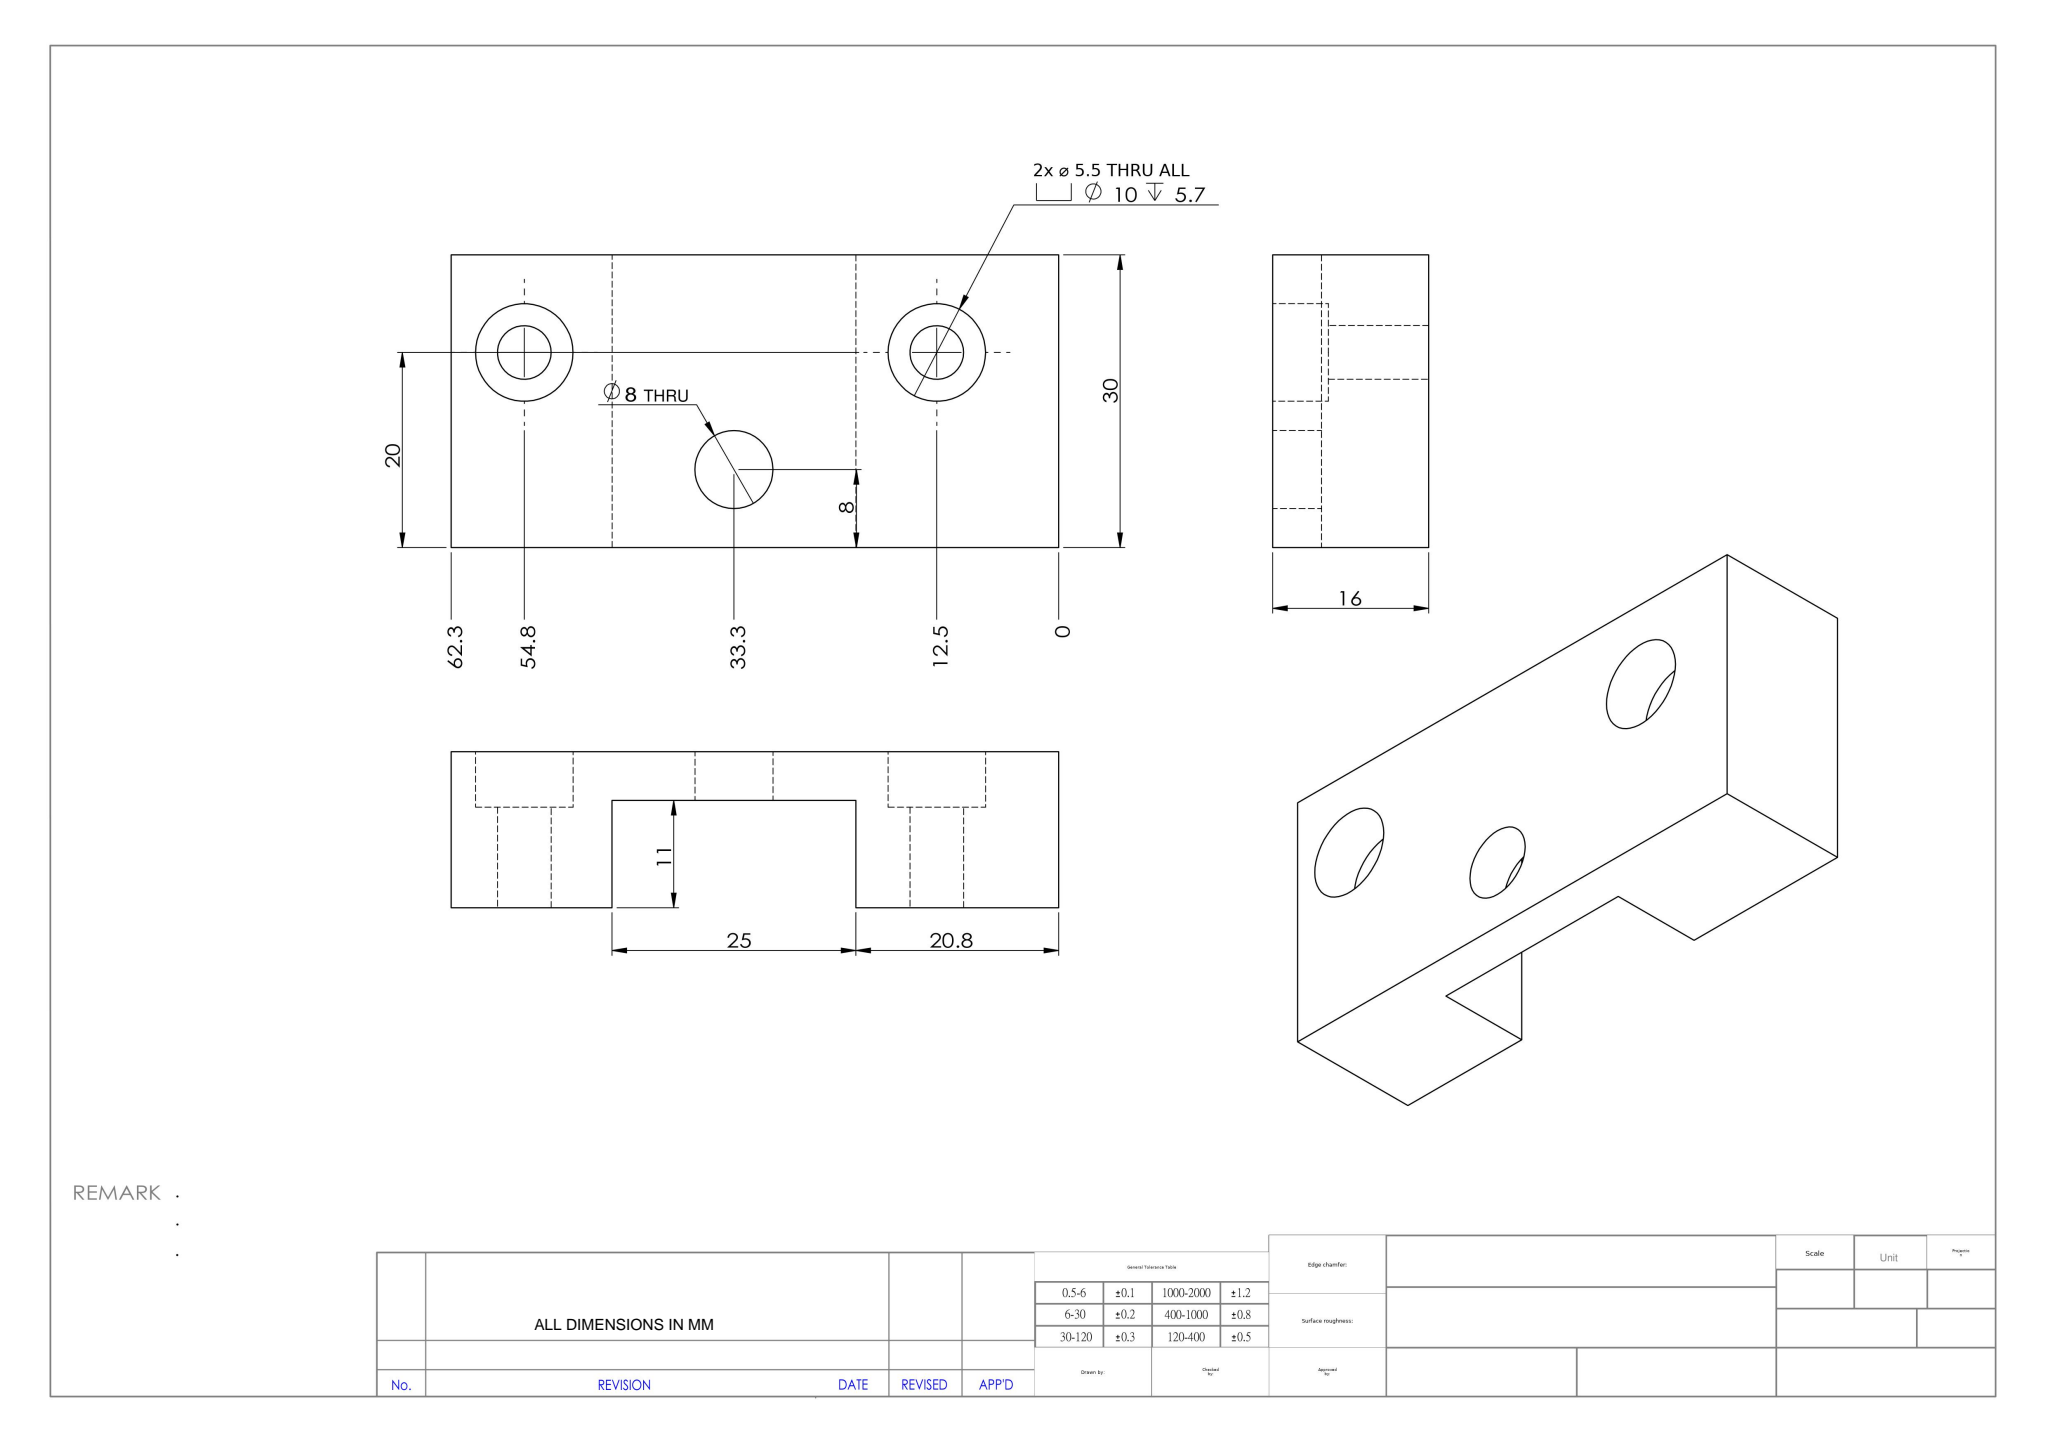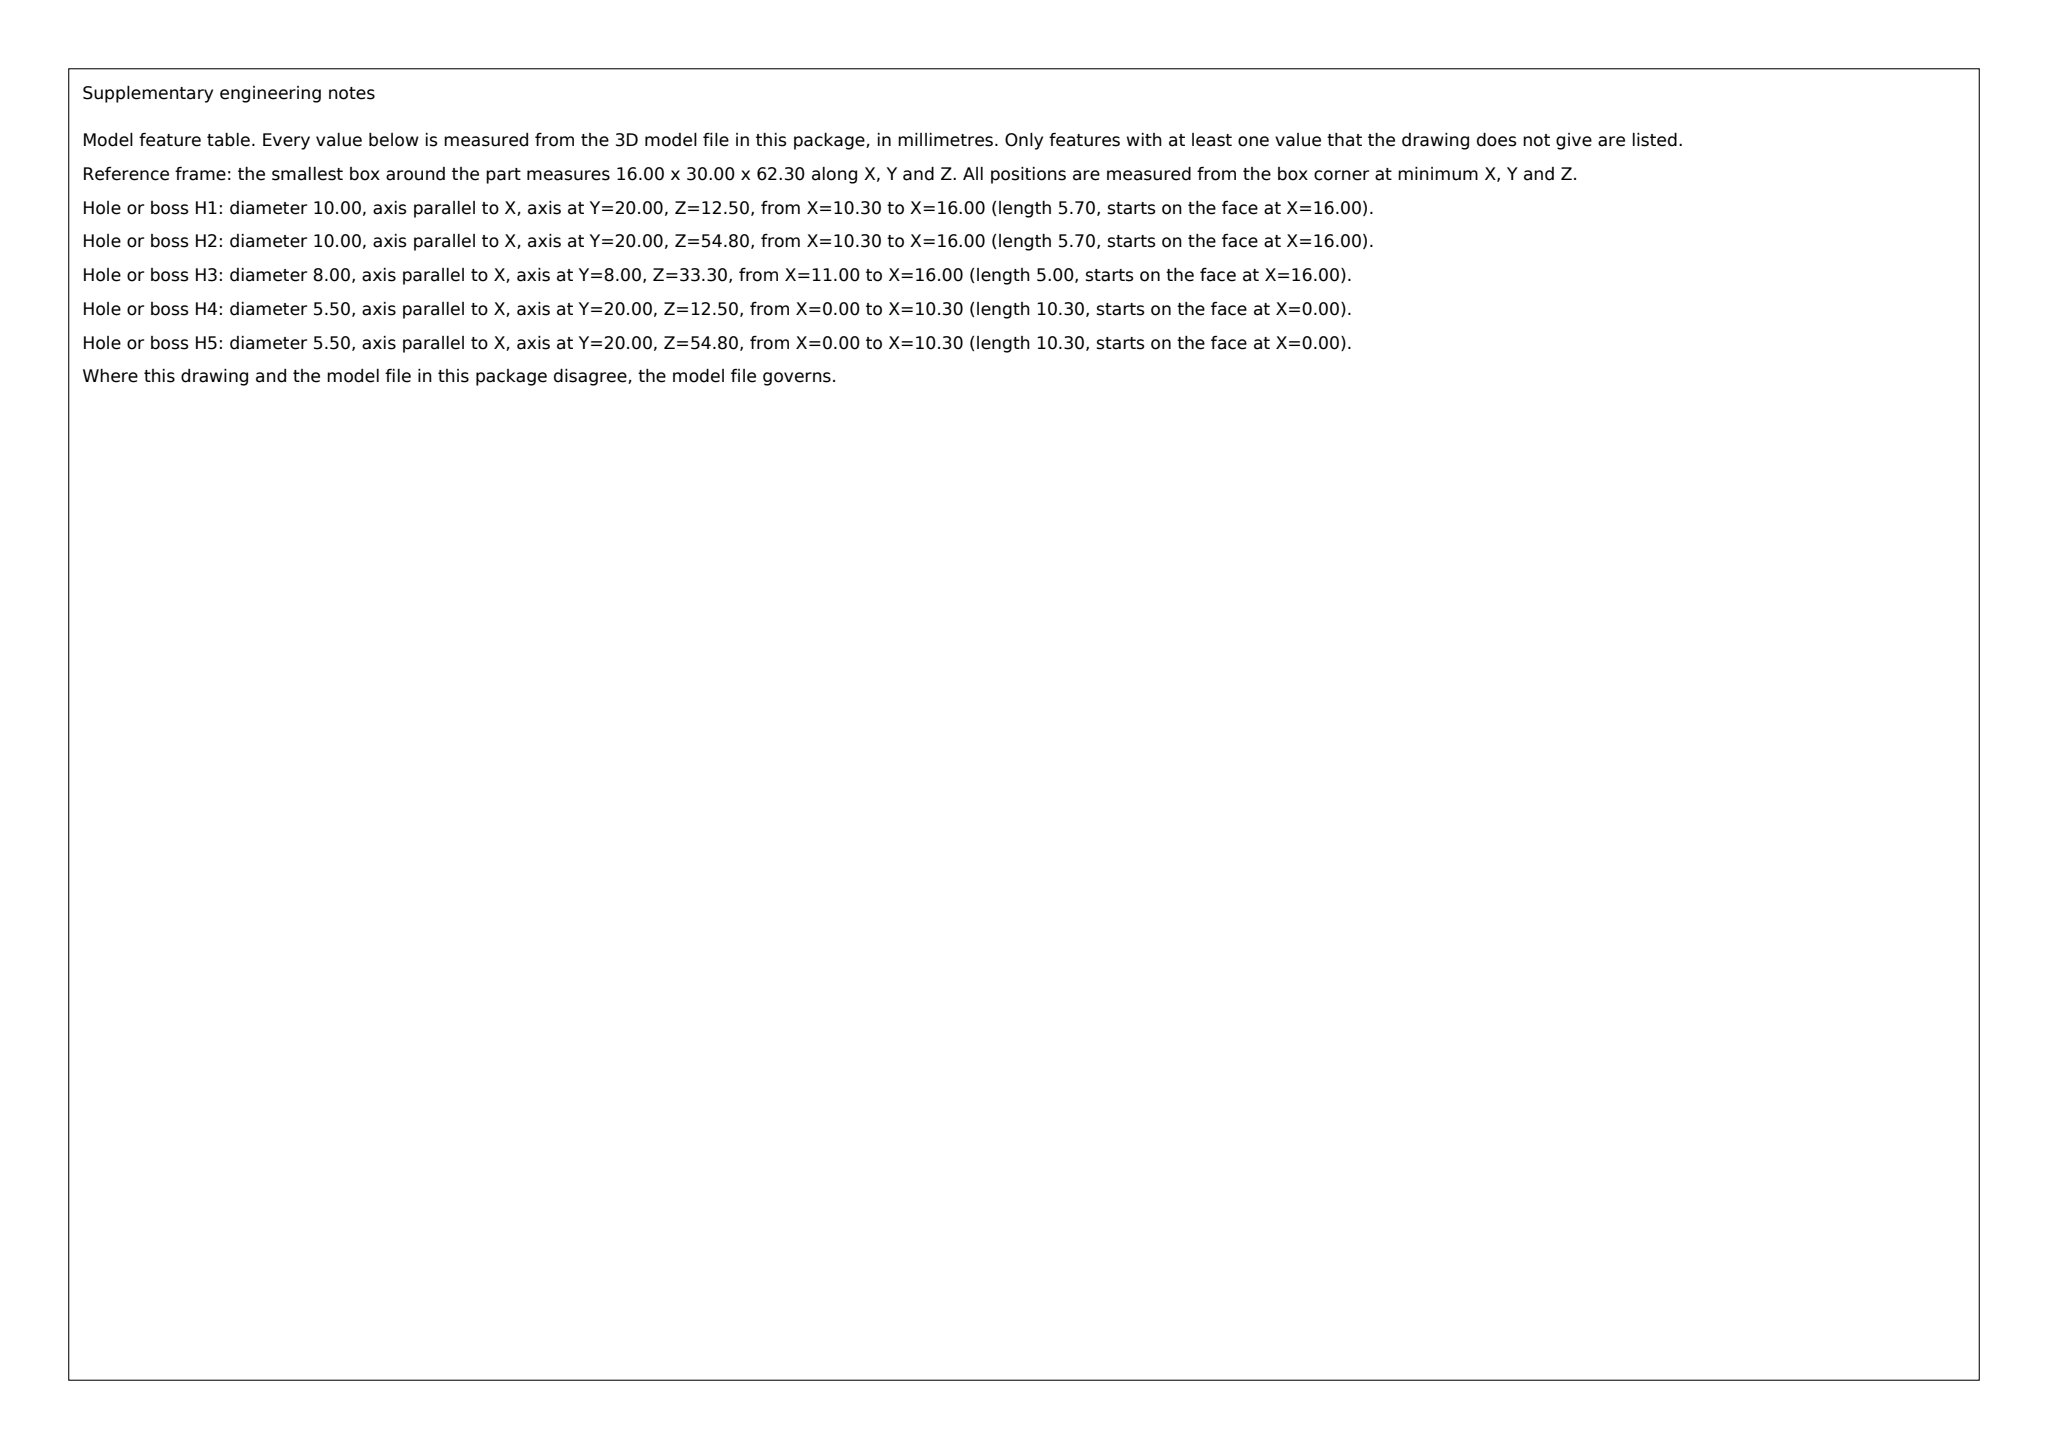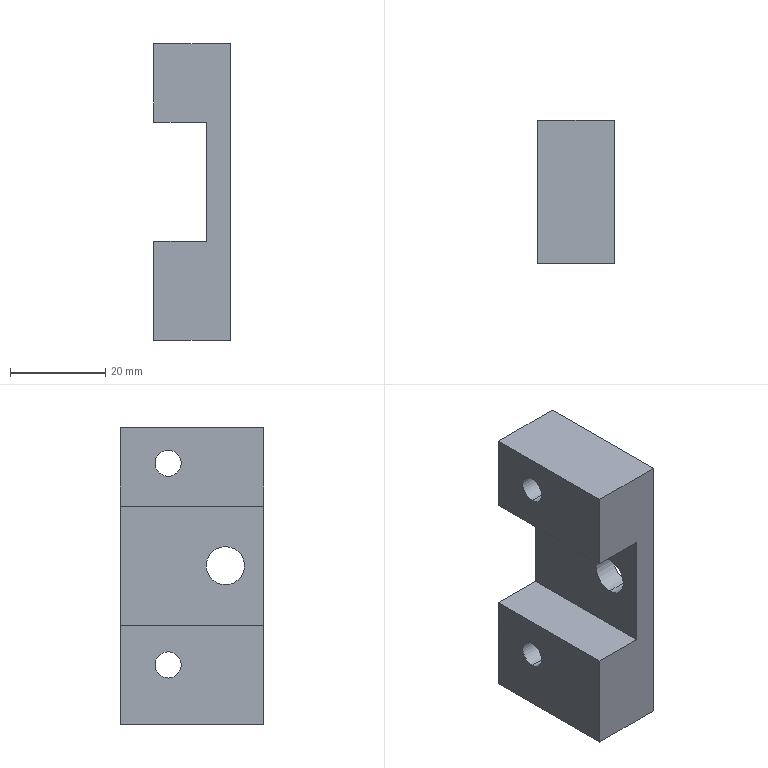Part | SolidWorks | mm | 1 solid | 22 faces | box 16 x 30 x 62.3 mm | volume 20018 mm3 | plane 12 | cylinder 10 | commonest cylinder face diameters 10 x4 5.5 x4 8 x2
build123d program:
from build123d import *

# Parameters (mm, degrees)
SKETCH1_W                                         = 62.3
SKETCH1_H                                         = 20
BOSS_EXTRUDE1_DEPTH                               = 16
HOLE_SIZE_ACCORDING_TO_TYPE_1_HEXAGON_D           = 5.5
HOLE_SIZE_ACCORDING_TO_TYPE_1_HEXAGON_CBORE_D     = 10
HOLE_SIZE_ACCORDING_TO_TYPE_1_HEXAGON_CBORE_DEPTH = 5.7
SKETCH5_W                                         = 16
SKETCH5_H                                         = 62.3
BOSS_EXTRUDE2_DEPTH                               = 10
SKETCH6_R                                         = 4
CUT_EXTRUDE1_DEPTH                                = 41.328
SKETCH7_W                                         = 25
SKETCH7_H                                         = 30
CUT_EXTRUDE2_DEPTH                                = 11


with BuildPart() as part:
    # Sketch1 → Boss-Extrude1 (new body)
    with BuildSketch(Plane(origin=(0, 0, 0), x_dir=(0, 0, -1), z_dir=(1, 0, 0))):
        Rectangle(SKETCH1_W, SKETCH1_H)
    extrude(amount=BOSS_EXTRUDE1_DEPTH)

    # Hole Size _ according to_ Type 1 Hexagon (through all)
    with Locations(Plane(origin=(16, 0, 0), x_dir=(0, 0, -1), z_dir=(1, 0, 0))):
        with Locations((-23.65, 0), (18.65, 0)):
            CounterBoreHole(HOLE_SIZE_ACCORDING_TO_TYPE_1_HEXAGON_D / 2, HOLE_SIZE_ACCORDING_TO_TYPE_1_HEXAGON_CBORE_D / 2, HOLE_SIZE_ACCORDING_TO_TYPE_1_HEXAGON_CBORE_DEPTH)

    # Sketch5 → Boss-Extrude2 (add)
    with BuildSketch(Plane.XZ.offset(10)):
        with Locations((8, 0)):
            Rectangle(SKETCH5_W, SKETCH5_H)
    extrude(amount=BOSS_EXTRUDE2_DEPTH)

    # Sketch6 → Cut-Extrude1 (cut, through all)
    with BuildSketch(Plane(origin=(16, 0, 0), x_dir=(0, 0, -1), z_dir=(1, 0, 0))):
        with Locations((-2.15, -12)):
            Circle(SKETCH6_R)
    extrude(amount=-CUT_EXTRUDE1_DEPTH, mode=Mode.SUBTRACT)

    # Sketch7 → Cut-Extrude2 (cut)
    with BuildSketch(Plane.ZY):
        with Locations((2.15, -5)):
            Rectangle(SKETCH7_W, SKETCH7_H)
    extrude(amount=-CUT_EXTRUDE2_DEPTH, mode=Mode.SUBTRACT)


solid = part.part
STEP:
#1=CARTESIAN_POINT('',(11.,-12.,-1.85));
#2=VERTEX_POINT('',#1);
#3=CARTESIAN_POINT('',(11.,-12.,6.15));
#4=VERTEX_POINT('',#3);
#5=CARTESIAN_POINT('',(11.,-12.,2.15));
#6=DIRECTION('',(-1.,0.,0.));
#7=DIRECTION('',(0.,0.,-1.));
#8=AXIS2_PLACEMENT_3D('',#5,#6,#7);
#9=CIRCLE('',#8,4.);
#10=EDGE_CURVE('',#2,#4,#9,.T.);
#11=ORIENTED_EDGE('',*,*,#10,.T.);
#12=CARTESIAN_POINT('',(16.,-12.,6.15));
#13=VERTEX_POINT('',#12);
#14=CARTESIAN_POINT('',(0.,-12.,6.15));
#15=DIRECTION('',(1.,0.,0.));
#16=VECTOR('',#15,1000.);
#17=LINE('',#14,#16);
#18=EDGE_CURVE('',#4,#13,#17,.T.);
#19=ORIENTED_EDGE('',*,*,#18,.T.);
#20=CARTESIAN_POINT('',(16.,-12.,-1.85));
#21=VERTEX_POINT('',#20);
#22=CARTESIAN_POINT('',(16.,-12.,2.15));
#23=DIRECTION('',(1.,0.,0.));
#24=DIRECTION('',(0.,0.,-1.));
#25=AXIS2_PLACEMENT_3D('',#22,#23,#24);
#26=CIRCLE('',#25,4.);
#27=EDGE_CURVE('',#13,#21,#26,.T.);
#28=ORIENTED_EDGE('',*,*,#27,.T.);
#29=CARTESIAN_POINT('',(0.,-12.,-1.85));
#30=DIRECTION('',(1.,0.,0.));
#31=VECTOR('',#30,1000.);
#32=LINE('',#29,#31);
#33=EDGE_CURVE('',#2,#21,#32,.T.);
#34=ORIENTED_EDGE('',*,*,#33,.F.);
#35=EDGE_LOOP('',(#11,#19,#28,#34));
#36=FACE_OUTER_BOUND('',#35,.T.);
#37=CARTESIAN_POINT('',(0.,-12.,2.15));
#38=DIRECTION('',(1.,0.,0.));
#39=DIRECTION('',(0.,0.,-1.));
#40=AXIS2_PLACEMENT_3D('',#37,#38,#39);
#41=CYLINDRICAL_SURFACE('',#40,4.);
#42=ADVANCED_FACE('',(#36),#41,.F.);
#43=CARTESIAN_POINT('',(10.3,0.,28.65));
#44=VERTEX_POINT('',#43);
#45=CARTESIAN_POINT('',(10.3,0.,18.65));
#46=VERTEX_POINT('',#45);
#47=CARTESIAN_POINT('',(10.3,0.,23.65));
#48=DIRECTION('',(1.,0.,0.));
#49=DIRECTION('',(0.,0.,-1.));
#50=AXIS2_PLACEMENT_3D('',#47,#48,#49);
#51=CIRCLE('',#50,5.);
#52=EDGE_CURVE('',#44,#46,#51,.T.);
#53=ORIENTED_EDGE('',*,*,#52,.F.);
#54=CARTESIAN_POINT('',(16.,0.,28.65));
#55=VERTEX_POINT('',#54);
#56=CARTESIAN_POINT('',(16.,0.,28.65));
#57=DIRECTION('',(1.,0.,0.));
#58=VECTOR('',#57,1000.);
#59=LINE('',#56,#58);
#60=EDGE_CURVE('',#44,#55,#59,.T.);
#61=ORIENTED_EDGE('',*,*,#60,.T.);
#62=CARTESIAN_POINT('',(16.,0.,18.65));
#63=VERTEX_POINT('',#62);
#64=CARTESIAN_POINT('',(16.,0.,23.65));
#65=DIRECTION('',(1.,0.,0.));
#66=DIRECTION('',(0.,0.,-1.));
#67=AXIS2_PLACEMENT_3D('',#64,#65,#66);
#68=CIRCLE('',#67,5.);
#69=EDGE_CURVE('',#55,#63,#68,.T.);
#70=ORIENTED_EDGE('',*,*,#69,.T.);
#71=CARTESIAN_POINT('',(16.,0.,18.65));
#72=DIRECTION('',(1.,0.,0.));
#73=VECTOR('',#72,1000.);
#74=LINE('',#71,#73);
#75=EDGE_CURVE('',#46,#63,#74,.T.);
#76=ORIENTED_EDGE('',*,*,#75,.F.);
#77=EDGE_LOOP('',(#53,#61,#70,#76));
#78=FACE_OUTER_BOUND('',#77,.T.);
#79=CARTESIAN_POINT('',(16.,0.,23.65));
#80=DIRECTION('',(1.,0.,0.));
#81=DIRECTION('',(0.,0.,-1.));
#82=AXIS2_PLACEMENT_3D('',#79,#80,#81);
#83=CYLINDRICAL_SURFACE('',#82,5.);
#84=ADVANCED_FACE('',(#78),#83,.F.);
#85=CARTESIAN_POINT('',(0.,0.,26.4));
#86=VERTEX_POINT('',#85);
#87=CARTESIAN_POINT('',(0.,0.,20.9));
#88=VERTEX_POINT('',#87);
#89=CARTESIAN_POINT('',(0.,0.,23.65));
#90=DIRECTION('',(1.,0.,0.));
#91=DIRECTION('',(0.,0.,-1.));
#92=AXIS2_PLACEMENT_3D('',#89,#90,#91);
#93=CIRCLE('',#92,2.75);
#94=EDGE_CURVE('',#86,#88,#93,.T.);
#95=ORIENTED_EDGE('',*,*,#94,.F.);
#96=CARTESIAN_POINT('',(10.3,0.,26.4));
#97=VERTEX_POINT('',#96);
#98=CARTESIAN_POINT('',(16.,0.,26.4));
#99=DIRECTION('',(1.,0.,0.));
#100=VECTOR('',#99,1000.);
#101=LINE('',#98,#100);
#102=EDGE_CURVE('',#86,#97,#101,.T.);
#103=ORIENTED_EDGE('',*,*,#102,.T.);
#104=CARTESIAN_POINT('',(10.3,0.,20.9));
#105=VERTEX_POINT('',#104);
#106=CARTESIAN_POINT('',(10.3,0.,23.65));
#107=DIRECTION('',(1.,0.,0.));
#108=DIRECTION('',(0.,0.,-1.));
#109=AXIS2_PLACEMENT_3D('',#106,#107,#108);
#110=CIRCLE('',#109,2.75);
#111=EDGE_CURVE('',#97,#105,#110,.T.);
#112=ORIENTED_EDGE('',*,*,#111,.T.);
#113=CARTESIAN_POINT('',(16.,0.,20.9));
#114=DIRECTION('',(1.,0.,0.));
#115=VECTOR('',#114,1000.);
#116=LINE('',#113,#115);
#117=EDGE_CURVE('',#88,#105,#116,.T.);
#118=ORIENTED_EDGE('',*,*,#117,.F.);
#119=EDGE_LOOP('',(#95,#103,#112,#118));
#120=FACE_OUTER_BOUND('',#119,.T.);
#121=CARTESIAN_POINT('',(16.,0.,23.65));
#122=DIRECTION('',(1.,0.,0.));
#123=DIRECTION('',(0.,0.,-1.));
#124=AXIS2_PLACEMENT_3D('',#121,#122,#123);
#125=CYLINDRICAL_SURFACE('',#124,2.75);
#126=ADVANCED_FACE('',(#120),#125,.F.);
#127=CARTESIAN_POINT('',(10.3,0.,-13.65));
#128=VERTEX_POINT('',#127);
#129=CARTESIAN_POINT('',(10.3,0.,-23.65));
#130=VERTEX_POINT('',#129);
#131=CARTESIAN_POINT('',(10.3,0.,-18.65));
#132=DIRECTION('',(1.,0.,0.));
#133=DIRECTION('',(0.,0.,-1.));
#134=AXIS2_PLACEMENT_3D('',#131,#132,#133);
#135=CIRCLE('',#134,5.);
#136=EDGE_CURVE('',#128,#130,#135,.T.);
#137=ORIENTED_EDGE('',*,*,#136,.F.);
#138=CARTESIAN_POINT('',(16.,0.,-13.65));
#139=VERTEX_POINT('',#138);
#140=CARTESIAN_POINT('',(16.,0.,-13.65));
#141=DIRECTION('',(1.,0.,0.));
#142=VECTOR('',#141,1000.);
#143=LINE('',#140,#142);
#144=EDGE_CURVE('',#128,#139,#143,.T.);
#145=ORIENTED_EDGE('',*,*,#144,.T.);
#146=CARTESIAN_POINT('',(16.,0.,-23.65));
#147=VERTEX_POINT('',#146);
#148=CARTESIAN_POINT('',(16.,0.,-18.65));
#149=DIRECTION('',(1.,0.,0.));
#150=DIRECTION('',(0.,0.,-1.));
#151=AXIS2_PLACEMENT_3D('',#148,#149,#150);
#152=CIRCLE('',#151,5.);
#153=EDGE_CURVE('',#139,#147,#152,.T.);
#154=ORIENTED_EDGE('',*,*,#153,.T.);
#155=CARTESIAN_POINT('',(16.,0.,-23.65));
#156=DIRECTION('',(1.,0.,0.));
#157=VECTOR('',#156,1000.);
#158=LINE('',#155,#157);
#159=EDGE_CURVE('',#130,#147,#158,.T.);
#160=ORIENTED_EDGE('',*,*,#159,.F.);
#161=EDGE_LOOP('',(#137,#145,#154,#160));
#162=FACE_OUTER_BOUND('',#161,.T.);
#163=CARTESIAN_POINT('',(16.,0.,-18.65));
#164=DIRECTION('',(1.,0.,0.));
#165=DIRECTION('',(0.,0.,-1.));
#166=AXIS2_PLACEMENT_3D('',#163,#164,#165);
#167=CYLINDRICAL_SURFACE('',#166,5.);
#168=ADVANCED_FACE('',(#162),#167,.F.);
#169=CARTESIAN_POINT('',(0.,0.,-15.9));
#170=VERTEX_POINT('',#169);
#171=CARTESIAN_POINT('',(0.,0.,-21.4));
#172=VERTEX_POINT('',#171);
#173=CARTESIAN_POINT('',(0.,0.,-18.65));
#174=DIRECTION('',(1.,0.,0.));
#175=DIRECTION('',(0.,0.,-1.));
#176=AXIS2_PLACEMENT_3D('',#173,#174,#175);
#177=CIRCLE('',#176,2.75);
#178=EDGE_CURVE('',#170,#172,#177,.T.);
#179=ORIENTED_EDGE('',*,*,#178,.F.);
#180=CARTESIAN_POINT('',(10.3,0.,-15.9));
#181=VERTEX_POINT('',#180);
#182=CARTESIAN_POINT('',(16.,0.,-15.9));
#183=DIRECTION('',(1.,0.,0.));
#184=VECTOR('',#183,1000.);
#185=LINE('',#182,#184);
#186=EDGE_CURVE('',#170,#181,#185,.T.);
#187=ORIENTED_EDGE('',*,*,#186,.T.);
#188=CARTESIAN_POINT('',(10.3,0.,-21.4));
#189=VERTEX_POINT('',#188);
#190=CARTESIAN_POINT('',(10.3,0.,-18.65));
#191=DIRECTION('',(1.,0.,0.));
#192=DIRECTION('',(0.,0.,-1.));
#193=AXIS2_PLACEMENT_3D('',#190,#191,#192);
#194=CIRCLE('',#193,2.75);
#195=EDGE_CURVE('',#181,#189,#194,.T.);
#196=ORIENTED_EDGE('',*,*,#195,.T.);
#197=CARTESIAN_POINT('',(16.,0.,-21.4));
#198=DIRECTION('',(1.,0.,0.));
#199=VECTOR('',#198,1000.);
#200=LINE('',#197,#199);
#201=EDGE_CURVE('',#172,#189,#200,.T.);
#202=ORIENTED_EDGE('',*,*,#201,.F.);
#203=EDGE_LOOP('',(#179,#187,#196,#202));
#204=FACE_OUTER_BOUND('',#203,.T.);
#205=CARTESIAN_POINT('',(16.,0.,-18.65));
#206=DIRECTION('',(1.,0.,0.));
#207=DIRECTION('',(0.,0.,-1.));
#208=AXIS2_PLACEMENT_3D('',#205,#206,#207);
#209=CYLINDRICAL_SURFACE('',#208,2.75);
#210=ADVANCED_FACE('',(#204),#209,.F.);
#211=CARTESIAN_POINT('',(0.,0.,-18.65));
#212=DIRECTION('',(1.,0.,0.));
#213=DIRECTION('',(0.,0.,-1.));
#214=AXIS2_PLACEMENT_3D('',#211,#212,#213);
#215=CIRCLE('',#214,2.75);
#216=EDGE_CURVE('',#172,#170,#215,.T.);
#217=ORIENTED_EDGE('',*,*,#216,.T.);
#218=ORIENTED_EDGE('',*,*,#178,.T.);
#219=EDGE_LOOP('',(#217,#218));
#220=FACE_BOUND('',#219,.T.);
#221=CARTESIAN_POINT('',(0.,-20.,-10.35));
#222=VERTEX_POINT('',#221);
#223=CARTESIAN_POINT('',(0.,-20.,-31.15));
#224=VERTEX_POINT('',#223);
#225=CARTESIAN_POINT('',(0.,-20.,31.15));
#226=DIRECTION('',(0.,0.,-1.));
#227=VECTOR('',#226,1000.);
#228=LINE('',#225,#227);
#229=EDGE_CURVE('',#222,#224,#228,.T.);
#230=ORIENTED_EDGE('',*,*,#229,.F.);
#231=CARTESIAN_POINT('',(0.,10.,-10.35));
#232=VERTEX_POINT('',#231);
#233=CARTESIAN_POINT('',(0.,-20.,-10.35));
#234=DIRECTION('',(0.,-1.,0.));
#235=VECTOR('',#234,1000.);
#236=LINE('',#233,#235);
#237=EDGE_CURVE('',#232,#222,#236,.T.);
#238=ORIENTED_EDGE('',*,*,#237,.F.);
#239=CARTESIAN_POINT('',(0.,10.,-31.15));
#240=VERTEX_POINT('',#239);
#241=CARTESIAN_POINT('',(0.,10.,-31.15));
#242=DIRECTION('',(0.,-0.,1.));
#243=VECTOR('',#242,1000.);
#244=LINE('',#241,#243);
#245=EDGE_CURVE('',#240,#232,#244,.T.);
#246=ORIENTED_EDGE('',*,*,#245,.F.);
#247=CARTESIAN_POINT('',(0.,-10.,-31.15));
#248=DIRECTION('',(0.,1.,0.));
#249=VECTOR('',#248,1000.);
#250=LINE('',#247,#249);
#251=EDGE_CURVE('',#224,#240,#250,.T.);
#252=ORIENTED_EDGE('',*,*,#251,.F.);
#253=EDGE_LOOP('',(#230,#238,#246,#252));
#254=FACE_OUTER_BOUND('',#253,.T.);
#255=CARTESIAN_POINT('',(0.,0.,0.));
#256=DIRECTION('',(1.,0.,0.));
#257=DIRECTION('',(0.,0.,-1.));
#258=AXIS2_PLACEMENT_3D('',#255,#256,#257);
#259=PLANE('',#258);
#260=ADVANCED_FACE('',(#220,#254),#259,.F.);
#261=CARTESIAN_POINT('',(0.,10.,31.15));
#262=VERTEX_POINT('',#261);
#263=CARTESIAN_POINT('',(0.,-20.,31.15));
#264=VERTEX_POINT('',#263);
#265=CARTESIAN_POINT('',(0.,-10.,31.15));
#266=DIRECTION('',(0.,-1.,0.));
#267=VECTOR('',#266,1000.);
#268=LINE('',#265,#267);
#269=EDGE_CURVE('',#262,#264,#268,.T.);
#270=ORIENTED_EDGE('',*,*,#269,.T.);
#271=CARTESIAN_POINT('',(16.,-20.,31.15));
#272=VERTEX_POINT('',#271);
#273=CARTESIAN_POINT('',(16.,-20.,31.15));
#274=DIRECTION('',(-1.,0.,0.));
#275=VECTOR('',#274,1000.);
#276=LINE('',#273,#275);
#277=EDGE_CURVE('',#272,#264,#276,.T.);
#278=ORIENTED_EDGE('',*,*,#277,.F.);
#279=CARTESIAN_POINT('',(16.,10.,31.15));
#280=VERTEX_POINT('',#279);
#281=CARTESIAN_POINT('',(16.,-10.,31.15));
#282=DIRECTION('',(0.,-1.,0.));
#283=VECTOR('',#282,1000.);
#284=LINE('',#281,#283);
#285=EDGE_CURVE('',#280,#272,#284,.T.);
#286=ORIENTED_EDGE('',*,*,#285,.F.);
#287=CARTESIAN_POINT('',(16.,10.,31.15));
#288=DIRECTION('',(-1.,0.,0.));
#289=VECTOR('',#288,1000.);
#290=LINE('',#287,#289);
#291=EDGE_CURVE('',#280,#262,#290,.T.);
#292=ORIENTED_EDGE('',*,*,#291,.T.);
#293=EDGE_LOOP('',(#270,#278,#286,#292));
#294=FACE_OUTER_BOUND('',#293,.T.);
#295=CARTESIAN_POINT('',(16.,-10.,31.15));
#296=DIRECTION('',(0.,0.,-1.));
#297=DIRECTION('',(-1.,0.,0.));
#298=AXIS2_PLACEMENT_3D('',#295,#296,#297);
#299=PLANE('',#298);
#300=ADVANCED_FACE('',(#294),#299,.F.);
#301=ORIENTED_EDGE('',*,*,#251,.T.);
#302=CARTESIAN_POINT('',(16.,10.,-31.15));
#303=VERTEX_POINT('',#302);
#304=CARTESIAN_POINT('',(16.,10.,-31.15));
#305=DIRECTION('',(-1.,0.,0.));
#306=VECTOR('',#305,1000.);
#307=LINE('',#304,#306);
#308=EDGE_CURVE('',#303,#240,#307,.T.);
#309=ORIENTED_EDGE('',*,*,#308,.F.);
#310=CARTESIAN_POINT('',(16.,-20.,-31.15));
#311=VERTEX_POINT('',#310);
#312=CARTESIAN_POINT('',(16.,-10.,-31.15));
#313=DIRECTION('',(0.,1.,0.));
#314=VECTOR('',#313,1000.);
#315=LINE('',#312,#314);
#316=EDGE_CURVE('',#311,#303,#315,.T.);
#317=ORIENTED_EDGE('',*,*,#316,.F.);
#318=CARTESIAN_POINT('',(0.,-20.,-31.15));
#319=DIRECTION('',(1.,0.,0.));
#320=VECTOR('',#319,1000.);
#321=LINE('',#318,#320);
#322=EDGE_CURVE('',#224,#311,#321,.T.);
#323=ORIENTED_EDGE('',*,*,#322,.F.);
#324=EDGE_LOOP('',(#301,#309,#317,#323));
#325=FACE_OUTER_BOUND('',#324,.T.);
#326=CARTESIAN_POINT('',(16.,-10.,-31.15));
#327=DIRECTION('',(0.,0.,1.));
#328=DIRECTION('',(1.,0.,0.));
#329=AXIS2_PLACEMENT_3D('',#326,#327,#328);
#330=PLANE('',#329);
#331=ADVANCED_FACE('',(#325),#330,.F.);
#332=ORIENTED_EDGE('',*,*,#245,.T.);
#333=CARTESIAN_POINT('',(11.,10.,-10.35));
#334=VERTEX_POINT('',#333);
#335=CARTESIAN_POINT('',(11.,10.,-10.35));
#336=DIRECTION('',(-1.,0.,0.));
#337=VECTOR('',#336,1000.);
#338=LINE('',#335,#337);
#339=EDGE_CURVE('',#334,#232,#338,.T.);
#340=ORIENTED_EDGE('',*,*,#339,.F.);
#341=CARTESIAN_POINT('',(11.,10.,14.65));
#342=VERTEX_POINT('',#341);
#343=CARTESIAN_POINT('',(11.,10.,-10.35));
#344=DIRECTION('',(0.,0.,-1.));
#345=VECTOR('',#344,1000.);
#346=LINE('',#343,#345);
#347=EDGE_CURVE('',#342,#334,#346,.T.);
#348=ORIENTED_EDGE('',*,*,#347,.F.);
#349=CARTESIAN_POINT('',(0.,10.,14.65));
#350=VERTEX_POINT('',#349);
#351=CARTESIAN_POINT('',(11.,10.,14.65));
#352=DIRECTION('',(-1.,0.,0.));
#353=VECTOR('',#352,1000.);
#354=LINE('',#351,#353);
#355=EDGE_CURVE('',#342,#350,#354,.T.);
#356=ORIENTED_EDGE('',*,*,#355,.T.);
#357=CARTESIAN_POINT('',(0.,10.,-31.15));
#358=DIRECTION('',(0.,-0.,1.));
#359=VECTOR('',#358,1000.);
#360=LINE('',#357,#359);
#361=EDGE_CURVE('',#350,#262,#360,.T.);
#362=ORIENTED_EDGE('',*,*,#361,.T.);
#363=ORIENTED_EDGE('',*,*,#291,.F.);
#364=CARTESIAN_POINT('',(16.,10.,-31.15));
#365=DIRECTION('',(0.,-0.,1.));
#366=VECTOR('',#365,1000.);
#367=LINE('',#364,#366);
#368=EDGE_CURVE('',#303,#280,#367,.T.);
#369=ORIENTED_EDGE('',*,*,#368,.F.);
#370=ORIENTED_EDGE('',*,*,#308,.T.);
#371=EDGE_LOOP('',(#332,#340,#348,#356,#362,#363,#369,#370));
#372=FACE_OUTER_BOUND('',#371,.T.);
#373=CARTESIAN_POINT('',(16.,10.,-31.15));
#374=DIRECTION('',(0.,-1.,-0.));
#375=DIRECTION('',(0.,0.,-1.));
#376=AXIS2_PLACEMENT_3D('',#373,#374,#375);
#377=PLANE('',#376);
#378=ADVANCED_FACE('',(#372),#377,.F.);
#379=CARTESIAN_POINT('',(16.,-12.,2.15));
#380=DIRECTION('',(1.,0.,0.));
#381=DIRECTION('',(0.,0.,-1.));
#382=AXIS2_PLACEMENT_3D('',#379,#380,#381);
#383=CIRCLE('',#382,4.);
#384=EDGE_CURVE('',#21,#13,#383,.T.);
#385=ORIENTED_EDGE('',*,*,#384,.F.);
#386=ORIENTED_EDGE('',*,*,#27,.F.);
#387=EDGE_LOOP('',(#385,#386));
#388=FACE_BOUND('',#387,.T.);
#389=CARTESIAN_POINT('',(16.,0.,23.65));
#390=DIRECTION('',(1.,0.,0.));
#391=DIRECTION('',(0.,0.,-1.));
#392=AXIS2_PLACEMENT_3D('',#389,#390,#391);
#393=CIRCLE('',#392,5.);
#394=EDGE_CURVE('',#63,#55,#393,.T.);
#395=ORIENTED_EDGE('',*,*,#394,.F.);
#396=ORIENTED_EDGE('',*,*,#69,.F.);
#397=EDGE_LOOP('',(#395,#396));
#398=FACE_BOUND('',#397,.T.);
#399=CARTESIAN_POINT('',(16.,0.,-18.65));
#400=DIRECTION('',(1.,0.,0.));
#401=DIRECTION('',(0.,0.,-1.));
#402=AXIS2_PLACEMENT_3D('',#399,#400,#401);
#403=CIRCLE('',#402,5.);
#404=EDGE_CURVE('',#147,#139,#403,.T.);
#405=ORIENTED_EDGE('',*,*,#404,.F.);
#406=ORIENTED_EDGE('',*,*,#153,.F.);
#407=EDGE_LOOP('',(#405,#406));
#408=FACE_BOUND('',#407,.T.);
#409=ORIENTED_EDGE('',*,*,#285,.T.);
#410=CARTESIAN_POINT('',(16.,-20.,-31.15));
#411=DIRECTION('',(0.,-0.,1.));
#412=VECTOR('',#411,1000.);
#413=LINE('',#410,#412);
#414=EDGE_CURVE('',#311,#272,#413,.T.);
#415=ORIENTED_EDGE('',*,*,#414,.F.);
#416=ORIENTED_EDGE('',*,*,#316,.T.);
#417=ORIENTED_EDGE('',*,*,#368,.T.);
#418=EDGE_LOOP('',(#409,#415,#416,#417));
#419=FACE_OUTER_BOUND('',#418,.T.);
#420=CARTESIAN_POINT('',(16.,0.,0.));
#421=DIRECTION('',(1.,0.,0.));
#422=DIRECTION('',(0.,0.,-1.));
#423=AXIS2_PLACEMENT_3D('',#420,#421,#422);
#424=PLANE('',#423);
#425=ADVANCED_FACE('',(#388,#398,#408,#419),#424,.T.);
#426=CARTESIAN_POINT('',(0.,0.,23.65));
#427=DIRECTION('',(1.,0.,0.));
#428=DIRECTION('',(0.,0.,-1.));
#429=AXIS2_PLACEMENT_3D('',#426,#427,#428);
#430=CIRCLE('',#429,2.75);
#431=EDGE_CURVE('',#88,#86,#430,.T.);
#432=ORIENTED_EDGE('',*,*,#431,.T.);
#433=ORIENTED_EDGE('',*,*,#94,.T.);
#434=EDGE_LOOP('',(#432,#433));
#435=FACE_BOUND('',#434,.T.);
#436=ORIENTED_EDGE('',*,*,#361,.F.);
#437=CARTESIAN_POINT('',(0.,-20.,14.65));
#438=VERTEX_POINT('',#437);
#439=CARTESIAN_POINT('',(0.,-20.,14.65));
#440=DIRECTION('',(0.,1.,0.));
#441=VECTOR('',#440,1000.);
#442=LINE('',#439,#441);
#443=EDGE_CURVE('',#438,#350,#442,.T.);
#444=ORIENTED_EDGE('',*,*,#443,.F.);
#445=CARTESIAN_POINT('',(0.,-20.,31.15));
#446=DIRECTION('',(0.,0.,-1.));
#447=VECTOR('',#446,1000.);
#448=LINE('',#445,#447);
#449=EDGE_CURVE('',#264,#438,#448,.T.);
#450=ORIENTED_EDGE('',*,*,#449,.F.);
#451=ORIENTED_EDGE('',*,*,#269,.F.);
#452=EDGE_LOOP('',(#436,#444,#450,#451));
#453=FACE_OUTER_BOUND('',#452,.T.);
#454=CARTESIAN_POINT('',(0.,0.,0.));
#455=DIRECTION('',(1.,0.,0.));
#456=DIRECTION('',(0.,0.,-1.));
#457=AXIS2_PLACEMENT_3D('',#454,#455,#456);
#458=PLANE('',#457);
#459=ADVANCED_FACE('',(#435,#453),#458,.F.);
#460=ORIENTED_EDGE('',*,*,#186,.F.);
#461=ORIENTED_EDGE('',*,*,#216,.F.);
#462=ORIENTED_EDGE('',*,*,#201,.T.);
#463=CARTESIAN_POINT('',(10.3,0.,-18.65));
#464=DIRECTION('',(1.,0.,0.));
#465=DIRECTION('',(0.,0.,-1.));
#466=AXIS2_PLACEMENT_3D('',#463,#464,#465);
#467=CIRCLE('',#466,2.75);
#468=EDGE_CURVE('',#189,#181,#467,.T.);
#469=ORIENTED_EDGE('',*,*,#468,.T.);
#470=EDGE_LOOP('',(#460,#461,#462,#469));
#471=FACE_OUTER_BOUND('',#470,.T.);
#472=CARTESIAN_POINT('',(16.,0.,-18.65));
#473=DIRECTION('',(1.,0.,0.));
#474=DIRECTION('',(0.,0.,-1.));
#475=AXIS2_PLACEMENT_3D('',#472,#473,#474);
#476=CYLINDRICAL_SURFACE('',#475,2.75);
#477=ADVANCED_FACE('',(#471),#476,.F.);
#478=ORIENTED_EDGE('',*,*,#468,.F.);
#479=ORIENTED_EDGE('',*,*,#195,.F.);
#480=EDGE_LOOP('',(#478,#479));
#481=FACE_BOUND('',#480,.T.);
#482=CARTESIAN_POINT('',(10.3,0.,-18.65));
#483=DIRECTION('',(1.,0.,0.));
#484=DIRECTION('',(0.,0.,-1.));
#485=AXIS2_PLACEMENT_3D('',#482,#483,#484);
#486=CIRCLE('',#485,5.);
#487=EDGE_CURVE('',#130,#128,#486,.T.);
#488=ORIENTED_EDGE('',*,*,#487,.T.);
#489=ORIENTED_EDGE('',*,*,#136,.T.);
#490=EDGE_LOOP('',(#488,#489));
#491=FACE_OUTER_BOUND('',#490,.T.);
#492=CARTESIAN_POINT('',(10.3,2.75,-18.65));
#493=DIRECTION('',(-1.,0.,0.));
#494=DIRECTION('',(0.,0.,1.));
#495=AXIS2_PLACEMENT_3D('',#492,#493,#494);
#496=PLANE('',#495);
#497=ADVANCED_FACE('',(#481,#491),#496,.F.);
#498=ORIENTED_EDGE('',*,*,#144,.F.);
#499=ORIENTED_EDGE('',*,*,#487,.F.);
#500=ORIENTED_EDGE('',*,*,#159,.T.);
#501=ORIENTED_EDGE('',*,*,#404,.T.);
#502=EDGE_LOOP('',(#498,#499,#500,#501));
#503=FACE_OUTER_BOUND('',#502,.T.);
#504=CARTESIAN_POINT('',(16.,0.,-18.65));
#505=DIRECTION('',(1.,0.,0.));
#506=DIRECTION('',(0.,0.,-1.));
#507=AXIS2_PLACEMENT_3D('',#504,#505,#506);
#508=CYLINDRICAL_SURFACE('',#507,5.);
#509=ADVANCED_FACE('',(#503),#508,.F.);
#510=ORIENTED_EDGE('',*,*,#102,.F.);
#511=ORIENTED_EDGE('',*,*,#431,.F.);
#512=ORIENTED_EDGE('',*,*,#117,.T.);
#513=CARTESIAN_POINT('',(10.3,0.,23.65));
#514=DIRECTION('',(1.,0.,0.));
#515=DIRECTION('',(0.,0.,-1.));
#516=AXIS2_PLACEMENT_3D('',#513,#514,#515);
#517=CIRCLE('',#516,2.75);
#518=EDGE_CURVE('',#105,#97,#517,.T.);
#519=ORIENTED_EDGE('',*,*,#518,.T.);
#520=EDGE_LOOP('',(#510,#511,#512,#519));
#521=FACE_OUTER_BOUND('',#520,.T.);
#522=CARTESIAN_POINT('',(16.,0.,23.65));
#523=DIRECTION('',(1.,0.,0.));
#524=DIRECTION('',(0.,0.,-1.));
#525=AXIS2_PLACEMENT_3D('',#522,#523,#524);
#526=CYLINDRICAL_SURFACE('',#525,2.75);
#527=ADVANCED_FACE('',(#521),#526,.F.);
#528=ORIENTED_EDGE('',*,*,#518,.F.);
#529=ORIENTED_EDGE('',*,*,#111,.F.);
#530=EDGE_LOOP('',(#528,#529));
#531=FACE_BOUND('',#530,.T.);
#532=CARTESIAN_POINT('',(10.3,0.,23.65));
#533=DIRECTION('',(1.,0.,0.));
#534=DIRECTION('',(0.,0.,-1.));
#535=AXIS2_PLACEMENT_3D('',#532,#533,#534);
#536=CIRCLE('',#535,5.);
#537=EDGE_CURVE('',#46,#44,#536,.T.);
#538=ORIENTED_EDGE('',*,*,#537,.T.);
#539=ORIENTED_EDGE('',*,*,#52,.T.);
#540=EDGE_LOOP('',(#538,#539));
#541=FACE_OUTER_BOUND('',#540,.T.);
#542=CARTESIAN_POINT('',(10.3,2.75,23.65));
#543=DIRECTION('',(-1.,0.,0.));
#544=DIRECTION('',(0.,0.,1.));
#545=AXIS2_PLACEMENT_3D('',#542,#543,#544);
#546=PLANE('',#545);
#547=ADVANCED_FACE('',(#531,#541),#546,.F.);
#548=ORIENTED_EDGE('',*,*,#60,.F.);
#549=ORIENTED_EDGE('',*,*,#537,.F.);
#550=ORIENTED_EDGE('',*,*,#75,.T.);
#551=ORIENTED_EDGE('',*,*,#394,.T.);
#552=EDGE_LOOP('',(#548,#549,#550,#551));
#553=FACE_OUTER_BOUND('',#552,.T.);
#554=CARTESIAN_POINT('',(16.,0.,23.65));
#555=DIRECTION('',(1.,0.,0.));
#556=DIRECTION('',(0.,0.,-1.));
#557=AXIS2_PLACEMENT_3D('',#554,#555,#556);
#558=CYLINDRICAL_SURFACE('',#557,5.);
#559=ADVANCED_FACE('',(#553),#558,.F.);
#560=CARTESIAN_POINT('',(11.,-20.,-10.35));
#561=VERTEX_POINT('',#560);
#562=CARTESIAN_POINT('',(11.,-20.,-10.35));
#563=DIRECTION('',(-1.,0.,0.));
#564=VECTOR('',#563,1000.);
#565=LINE('',#562,#564);
#566=EDGE_CURVE('',#561,#222,#565,.T.);
#567=ORIENTED_EDGE('',*,*,#566,.T.);
#568=ORIENTED_EDGE('',*,*,#229,.T.);
#569=ORIENTED_EDGE('',*,*,#322,.T.);
#570=ORIENTED_EDGE('',*,*,#414,.T.);
#571=ORIENTED_EDGE('',*,*,#277,.T.);
#572=ORIENTED_EDGE('',*,*,#449,.T.);
#573=CARTESIAN_POINT('',(11.,-20.,14.65));
#574=VERTEX_POINT('',#573);
#575=CARTESIAN_POINT('',(11.,-20.,14.65));
#576=DIRECTION('',(-1.,0.,0.));
#577=VECTOR('',#576,1000.);
#578=LINE('',#575,#577);
#579=EDGE_CURVE('',#574,#438,#578,.T.);
#580=ORIENTED_EDGE('',*,*,#579,.F.);
#581=CARTESIAN_POINT('',(11.,-20.,-10.35));
#582=DIRECTION('',(0.,0.,1.));
#583=VECTOR('',#582,1000.);
#584=LINE('',#581,#583);
#585=EDGE_CURVE('',#561,#574,#584,.T.);
#586=ORIENTED_EDGE('',*,*,#585,.F.);
#587=EDGE_LOOP('',(#567,#568,#569,#570,#571,#572,#580,#586));
#588=FACE_OUTER_BOUND('',#587,.T.);
#589=CARTESIAN_POINT('',(0.,-20.,-0.));
#590=DIRECTION('',(0.,-1.,-0.));
#591=DIRECTION('',(0.,0.,-1.));
#592=AXIS2_PLACEMENT_3D('',#589,#590,#591);
#593=PLANE('',#592);
#594=ADVANCED_FACE('',(#588),#593,.T.);
#595=ORIENTED_EDGE('',*,*,#18,.F.);
#596=CARTESIAN_POINT('',(11.,-12.,2.15));
#597=DIRECTION('',(-1.,0.,0.));
#598=DIRECTION('',(0.,0.,-1.));
#599=AXIS2_PLACEMENT_3D('',#596,#597,#598);
#600=CIRCLE('',#599,4.);
#601=EDGE_CURVE('',#4,#2,#600,.T.);
#602=ORIENTED_EDGE('',*,*,#601,.T.);
#603=ORIENTED_EDGE('',*,*,#33,.T.);
#604=ORIENTED_EDGE('',*,*,#384,.T.);
#605=EDGE_LOOP('',(#595,#602,#603,#604));
#606=FACE_OUTER_BOUND('',#605,.T.);
#607=CARTESIAN_POINT('',(0.,-12.,2.15));
#608=DIRECTION('',(1.,0.,0.));
#609=DIRECTION('',(0.,0.,-1.));
#610=AXIS2_PLACEMENT_3D('',#607,#608,#609);
#611=CYLINDRICAL_SURFACE('',#610,4.);
#612=ADVANCED_FACE('',(#606),#611,.F.);
#613=CARTESIAN_POINT('',(11.,-20.,-10.35));
#614=DIRECTION('',(0.,-1.,0.));
#615=VECTOR('',#614,1000.);
#616=LINE('',#613,#615);
#617=EDGE_CURVE('',#334,#561,#616,.T.);
#618=ORIENTED_EDGE('',*,*,#617,.T.);
#619=ORIENTED_EDGE('',*,*,#585,.T.);
#620=CARTESIAN_POINT('',(11.,-20.,14.65));
#621=DIRECTION('',(0.,1.,0.));
#622=VECTOR('',#621,1000.);
#623=LINE('',#620,#622);
#624=EDGE_CURVE('',#574,#342,#623,.T.);
#625=ORIENTED_EDGE('',*,*,#624,.T.);
#626=ORIENTED_EDGE('',*,*,#347,.T.);
#627=EDGE_LOOP('',(#618,#619,#625,#626));
#628=FACE_OUTER_BOUND('',#627,.T.);
#629=ORIENTED_EDGE('',*,*,#10,.F.);
#630=ORIENTED_EDGE('',*,*,#601,.F.);
#631=EDGE_LOOP('',(#629,#630));
#632=FACE_BOUND('',#631,.T.);
#633=CARTESIAN_POINT('',(11.,0.,0.));
#634=DIRECTION('',(1.,0.,0.));
#635=DIRECTION('',(0.,0.,-1.));
#636=AXIS2_PLACEMENT_3D('',#633,#634,#635);
#637=PLANE('',#636);
#638=ADVANCED_FACE('',(#628,#632),#637,.F.);
#639=ORIENTED_EDGE('',*,*,#237,.T.);
#640=ORIENTED_EDGE('',*,*,#566,.F.);
#641=ORIENTED_EDGE('',*,*,#617,.F.);
#642=ORIENTED_EDGE('',*,*,#339,.T.);
#643=EDGE_LOOP('',(#639,#640,#641,#642));
#644=FACE_OUTER_BOUND('',#643,.T.);
#645=CARTESIAN_POINT('',(11.,-20.,-10.35));
#646=DIRECTION('',(0.,0.,-1.));
#647=DIRECTION('',(-1.,0.,0.));
#648=AXIS2_PLACEMENT_3D('',#645,#646,#647);
#649=PLANE('',#648);
#650=ADVANCED_FACE('',(#644),#649,.F.);
#651=ORIENTED_EDGE('',*,*,#443,.T.);
#652=ORIENTED_EDGE('',*,*,#355,.F.);
#653=ORIENTED_EDGE('',*,*,#624,.F.);
#654=ORIENTED_EDGE('',*,*,#579,.T.);
#655=EDGE_LOOP('',(#651,#652,#653,#654));
#656=FACE_OUTER_BOUND('',#655,.T.);
#657=CARTESIAN_POINT('',(11.,-20.,14.65));
#658=DIRECTION('',(0.,0.,1.));
#659=DIRECTION('',(1.,0.,0.));
#660=AXIS2_PLACEMENT_3D('',#657,#658,#659);
#661=PLANE('',#660);
#662=ADVANCED_FACE('',(#656),#661,.F.);
#663=CLOSED_SHELL('',(#42,#84,#126,#168,#210,#260,#300,#331,#378,#425,#459,#477,#497,#509,#527,#547,#559,#594,#612,#638,#650,#662));
#664=MANIFOLD_SOLID_BREP('',#663);
#665=CARTESIAN_POINT('',(0.,0.,0.));
#666=DIRECTION('',(0.,0.,1.));
#667=DIRECTION('',(1.,0.,0.));
#668=AXIS2_PLACEMENT_3D('',#665,#666,#667);
#669=(LENGTH_UNIT()NAMED_UNIT(*)SI_UNIT(.MILLI.,.METRE.));
#670=UNCERTAINTY_MEASURE_WITH_UNIT(LENGTH_MEASURE(0.00001),#669,'','');
#671=(NAMED_UNIT(*)PLANE_ANGLE_UNIT()SI_UNIT($,.RADIAN.));
#672=(NAMED_UNIT(*)SI_UNIT($,.STERADIAN.)SOLID_ANGLE_UNIT());
#673=(GEOMETRIC_REPRESENTATION_CONTEXT(3)GLOBAL_UNCERTAINTY_ASSIGNED_CONTEXT((#670))GLOBAL_UNIT_ASSIGNED_CONTEXT((#669,#671,#672))REPRESENTATION_CONTEXT('',''));
#674=ADVANCED_BREP_SHAPE_REPRESENTATION('',(#664,#668),#673);